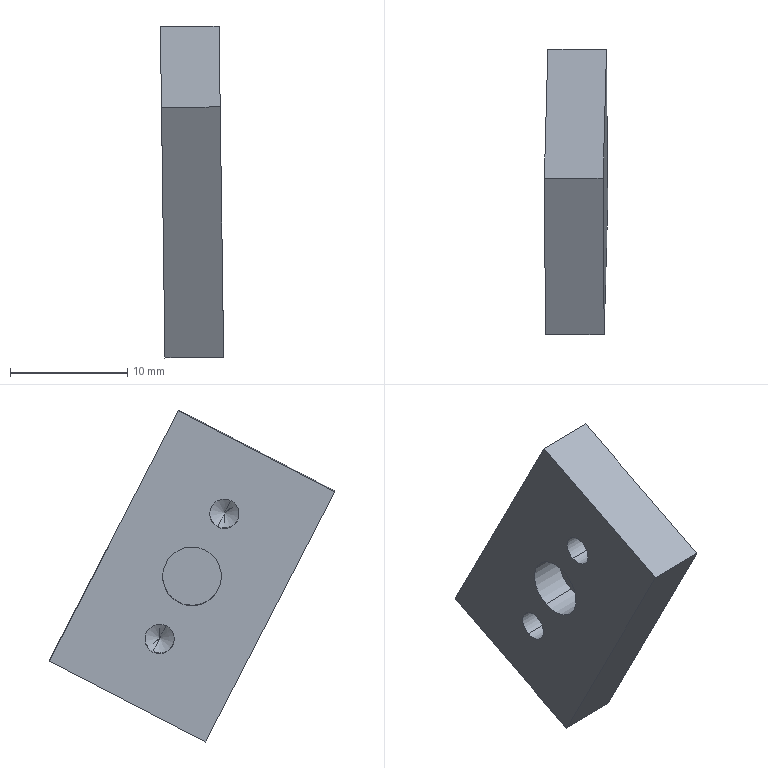Component | SolidWorks | 2018SOLIDWORKS1400000015-1 | 1 solid | 17 faces | box 5.39 x 24.34 x 28.27 mm | volume 1699 mm3 | plane 7 | cylinder 6 | cone 4 | commonest cylinder face diameters 2.5 x4 5 x2 | material 45 Steel
build123d program:
from build123d import *

# Parameters (mm, degrees)
SKETCH1_W             = 24
SKETCH1_H             = 15
BOSS_EXTRUDE1_DEPTH   = 5
M3_TAPPED_HOLE1_D     = 2.5
M3_TAPPED_HOLE1_DEPTH = 4
M3_TAPPED_HOLE1_TIP   = 0.7511
SKETCH4_R             = 2.5
CUT_EXTRUDE1_DEPTH    = 3


with BuildPart() as part:
    # Sketch1 → Boss-Extrude1 (new body)
    with BuildSketch(Plane.XY):
        Rectangle(SKETCH1_W, SKETCH1_H)
    extrude(amount=BOSS_EXTRUDE1_DEPTH)

    # M3 Tapped Hole1
    with Locations(Plane.XY.offset(5)):
        with Locations((-6, 0), (6, 0)):
            Hole(M3_TAPPED_HOLE1_D / 2, depth=M3_TAPPED_HOLE1_DEPTH)
            with Locations((0, 0, -(M3_TAPPED_HOLE1_DEPTH + M3_TAPPED_HOLE1_TIP / 2))):  # 118° drill point
                Cone(0, M3_TAPPED_HOLE1_D / 2, M3_TAPPED_HOLE1_TIP, mode=Mode.SUBTRACT)

    # Sketch4 → Cut-Extrude1 (cut)
    with BuildSketch(Plane.XY.offset(5)):
        Circle(SKETCH4_R)
    extrude(amount=-CUT_EXTRUDE1_DEPTH, mode=Mode.SUBTRACT)


solid = part.part

# Placed as in the assembly
solid = solid.moved(Location((87.559, -98.378, 177.073), (180, -89.207, 152.677)))